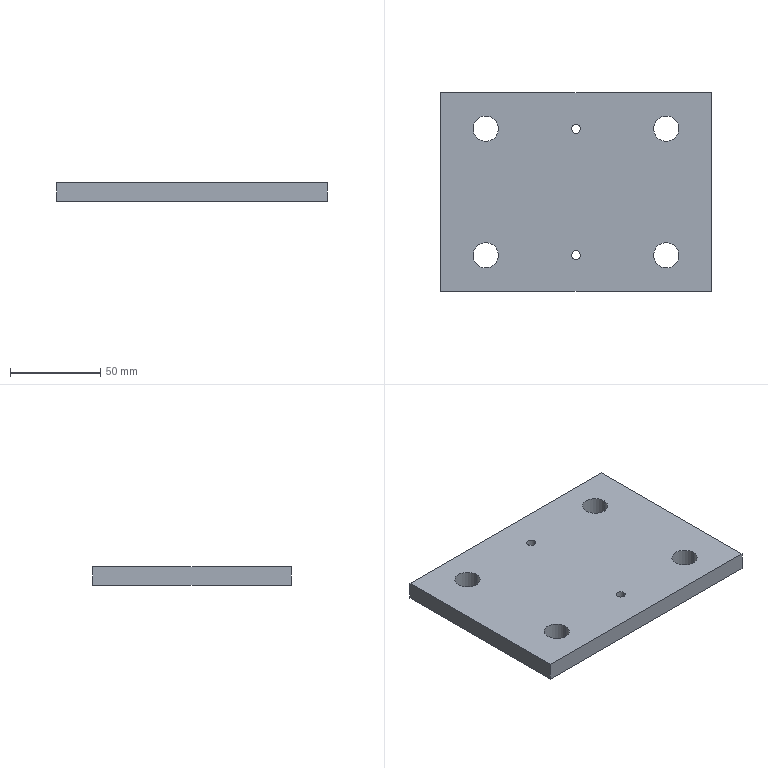Component | SolidWorks | THK-A1025ColumnFixingPlate-6 | 1 solid | 18 faces | box 150 x 110 x 10 mm | volume 158450 mm3 | cylinder 12 | plane 6 | commonest cylinder face diameters 14 x8 5 x4 | material Q235A
build123d program:
from build123d import *

# Parameters (mm, degrees)
SKETCH1_W                  = 150
SKETCH1_H                  = 110
BOSS_EXTRUDE1_DEPTH        = 5
F_14_0_14_DIAMETER_HOLE1_D = 14
M6_TAPPED_HOLE1_D          = 5


with BuildPart() as part:
    # Sketch1 → Boss-Extrude1 (new, symmetric)
    with BuildSketch(Plane.XY):
        Rectangle(SKETCH1_W, SKETCH1_H)
    extrude(amount=BOSS_EXTRUDE1_DEPTH, both=True)

    # 14.0 _14_ Diameter Hole1 (through all)
    with Locations(Plane.XY.offset(5)):
        with Locations((-50, 35), (50, 35), (50, -35), (-50, -35)):
            Hole(F_14_0_14_DIAMETER_HOLE1_D / 2)

    # M6 Tapped Hole1 (through all)
    with Locations(Plane.XY.offset(5)):
        with Locations((0, 35), (0, -35)):
            Hole(M6_TAPPED_HOLE1_D / 2)


solid = part.part

# Placed as in the assembly
solid = solid.moved(Location((0, 625, -376), (0, 0, 0)))
STEP:
#1=COLOUR_RGB('',0.7922,0.8196,0.9333);
#2=FILL_AREA_STYLE_COLOUR('',#1);
#3=FILL_AREA_STYLE('',(#2));
#4=SURFACE_STYLE_FILL_AREA(#3);
#5=SURFACE_SIDE_STYLE('',(#4));
#6=SURFACE_STYLE_USAGE(.BOTH.,#5);
#7=PRESENTATION_STYLE_ASSIGNMENT((#6));
#8=CARTESIAN_POINT('',(-0.09843,25.984,-15.));
#9=VERTEX_POINT('',#8);
#10=CARTESIAN_POINT('',(0.09843,25.984,-15.));
#11=VERTEX_POINT('',#10);
#12=CARTESIAN_POINT('',(0.,25.984,-15.));
#13=DIRECTION('',(0.,0.,1.));
#14=DIRECTION('',(1.,0.,0.));
#15=AXIS2_PLACEMENT_3D('',#12,#13,#14);
#16=CIRCLE('',#15,0.09843);
#17=EDGE_CURVE('',#9,#11,#16,.T.);
#18=ORIENTED_EDGE('',*,*,#17,.F.);
#19=CARTESIAN_POINT('',(-0.09843,25.984,-14.606));
#20=VERTEX_POINT('',#19);
#21=CARTESIAN_POINT('',(-0.09843,25.984,-14.606));
#22=DIRECTION('',(0.,0.,1.));
#23=VECTOR('',#22,39.37);
#24=LINE('',#21,#23);
#25=EDGE_CURVE('',#9,#20,#24,.T.);
#26=ORIENTED_EDGE('',*,*,#25,.T.);
#27=CARTESIAN_POINT('',(0.09843,25.984,-14.606));
#28=VERTEX_POINT('',#27);
#29=CARTESIAN_POINT('',(0.,25.984,-14.606));
#30=DIRECTION('',(0.,0.,1.));
#31=DIRECTION('',(1.,0.,0.));
#32=AXIS2_PLACEMENT_3D('',#29,#30,#31);
#33=CIRCLE('',#32,0.09843);
#34=EDGE_CURVE('',#20,#28,#33,.T.);
#35=ORIENTED_EDGE('',*,*,#34,.T.);
#36=CARTESIAN_POINT('',(0.09843,25.984,-14.606));
#37=DIRECTION('',(0.,0.,1.));
#38=VECTOR('',#37,39.37);
#39=LINE('',#36,#38);
#40=EDGE_CURVE('',#11,#28,#39,.T.);
#41=ORIENTED_EDGE('',*,*,#40,.F.);
#42=EDGE_LOOP('',(#18,#26,#35,#41));
#43=FACE_OUTER_BOUND('',#42,.T.);
#44=CARTESIAN_POINT('',(0.,25.984,-14.606));
#45=DIRECTION('',(0.,0.,1.));
#46=DIRECTION('',(1.,0.,0.));
#47=AXIS2_PLACEMENT_3D('',#44,#45,#46);
#48=CYLINDRICAL_SURFACE('',#47,0.09843);
#49=ADVANCED_FACE('',(#43),#48,.F.);
#50=CARTESIAN_POINT('',(-0.09843,23.228,-15.));
#51=VERTEX_POINT('',#50);
#52=CARTESIAN_POINT('',(0.09843,23.228,-15.));
#53=VERTEX_POINT('',#52);
#54=CARTESIAN_POINT('',(0.,23.228,-15.));
#55=DIRECTION('',(0.,0.,1.));
#56=DIRECTION('',(1.,0.,0.));
#57=AXIS2_PLACEMENT_3D('',#54,#55,#56);
#58=CIRCLE('',#57,0.09843);
#59=EDGE_CURVE('',#51,#53,#58,.T.);
#60=ORIENTED_EDGE('',*,*,#59,.F.);
#61=CARTESIAN_POINT('',(-0.09843,23.228,-14.606));
#62=VERTEX_POINT('',#61);
#63=CARTESIAN_POINT('',(-0.09843,23.228,-14.606));
#64=DIRECTION('',(0.,0.,1.));
#65=VECTOR('',#64,39.37);
#66=LINE('',#63,#65);
#67=EDGE_CURVE('',#51,#62,#66,.T.);
#68=ORIENTED_EDGE('',*,*,#67,.T.);
#69=CARTESIAN_POINT('',(0.09843,23.228,-14.606));
#70=VERTEX_POINT('',#69);
#71=CARTESIAN_POINT('',(0.,23.228,-14.606));
#72=DIRECTION('',(0.,0.,1.));
#73=DIRECTION('',(1.,0.,0.));
#74=AXIS2_PLACEMENT_3D('',#71,#72,#73);
#75=CIRCLE('',#74,0.09843);
#76=EDGE_CURVE('',#62,#70,#75,.T.);
#77=ORIENTED_EDGE('',*,*,#76,.T.);
#78=CARTESIAN_POINT('',(0.09843,23.228,-14.606));
#79=DIRECTION('',(0.,0.,1.));
#80=VECTOR('',#79,39.37);
#81=LINE('',#78,#80);
#82=EDGE_CURVE('',#53,#70,#81,.T.);
#83=ORIENTED_EDGE('',*,*,#82,.F.);
#84=EDGE_LOOP('',(#60,#68,#77,#83));
#85=FACE_OUTER_BOUND('',#84,.T.);
#86=CARTESIAN_POINT('',(0.,23.228,-14.606));
#87=DIRECTION('',(0.,0.,1.));
#88=DIRECTION('',(1.,0.,0.));
#89=AXIS2_PLACEMENT_3D('',#86,#87,#88);
#90=CYLINDRICAL_SURFACE('',#89,0.09843);
#91=ADVANCED_FACE('',(#85),#90,.F.);
#92=CARTESIAN_POINT('',(-2.244,25.984,-15.));
#93=VERTEX_POINT('',#92);
#94=CARTESIAN_POINT('',(-1.693,25.984,-15.));
#95=VERTEX_POINT('',#94);
#96=CARTESIAN_POINT('',(-1.969,25.984,-15.));
#97=DIRECTION('',(0.,0.,1.));
#98=DIRECTION('',(1.,0.,0.));
#99=AXIS2_PLACEMENT_3D('',#96,#97,#98);
#100=CIRCLE('',#99,0.2756);
#101=EDGE_CURVE('',#93,#95,#100,.T.);
#102=ORIENTED_EDGE('',*,*,#101,.F.);
#103=CARTESIAN_POINT('',(-2.244,25.984,-14.606));
#104=VERTEX_POINT('',#103);
#105=CARTESIAN_POINT('',(-2.244,25.984,-14.606));
#106=DIRECTION('',(0.,0.,1.));
#107=VECTOR('',#106,39.37);
#108=LINE('',#105,#107);
#109=EDGE_CURVE('',#93,#104,#108,.T.);
#110=ORIENTED_EDGE('',*,*,#109,.T.);
#111=CARTESIAN_POINT('',(-1.693,25.984,-14.606));
#112=VERTEX_POINT('',#111);
#113=CARTESIAN_POINT('',(-1.969,25.984,-14.606));
#114=DIRECTION('',(0.,0.,1.));
#115=DIRECTION('',(1.,0.,0.));
#116=AXIS2_PLACEMENT_3D('',#113,#114,#115);
#117=CIRCLE('',#116,0.2756);
#118=EDGE_CURVE('',#104,#112,#117,.T.);
#119=ORIENTED_EDGE('',*,*,#118,.T.);
#120=CARTESIAN_POINT('',(-1.693,25.984,-14.606));
#121=DIRECTION('',(0.,0.,1.));
#122=VECTOR('',#121,39.37);
#123=LINE('',#120,#122);
#124=EDGE_CURVE('',#95,#112,#123,.T.);
#125=ORIENTED_EDGE('',*,*,#124,.F.);
#126=EDGE_LOOP('',(#102,#110,#119,#125));
#127=FACE_OUTER_BOUND('',#126,.T.);
#128=CARTESIAN_POINT('',(-1.969,25.984,-14.606));
#129=DIRECTION('',(0.,0.,1.));
#130=DIRECTION('',(1.,0.,0.));
#131=AXIS2_PLACEMENT_3D('',#128,#129,#130);
#132=CYLINDRICAL_SURFACE('',#131,0.2756);
#133=ADVANCED_FACE('',(#127),#132,.F.);
#134=CARTESIAN_POINT('',(1.693,25.984,-15.));
#135=VERTEX_POINT('',#134);
#136=CARTESIAN_POINT('',(2.244,25.984,-15.));
#137=VERTEX_POINT('',#136);
#138=CARTESIAN_POINT('',(1.969,25.984,-15.));
#139=DIRECTION('',(0.,0.,1.));
#140=DIRECTION('',(1.,0.,0.));
#141=AXIS2_PLACEMENT_3D('',#138,#139,#140);
#142=CIRCLE('',#141,0.2756);
#143=EDGE_CURVE('',#135,#137,#142,.T.);
#144=ORIENTED_EDGE('',*,*,#143,.F.);
#145=CARTESIAN_POINT('',(1.693,25.984,-14.606));
#146=VERTEX_POINT('',#145);
#147=CARTESIAN_POINT('',(1.693,25.984,-14.606));
#148=DIRECTION('',(0.,0.,1.));
#149=VECTOR('',#148,39.37);
#150=LINE('',#147,#149);
#151=EDGE_CURVE('',#135,#146,#150,.T.);
#152=ORIENTED_EDGE('',*,*,#151,.T.);
#153=CARTESIAN_POINT('',(2.244,25.984,-14.606));
#154=VERTEX_POINT('',#153);
#155=CARTESIAN_POINT('',(1.969,25.984,-14.606));
#156=DIRECTION('',(0.,0.,1.));
#157=DIRECTION('',(1.,0.,0.));
#158=AXIS2_PLACEMENT_3D('',#155,#156,#157);
#159=CIRCLE('',#158,0.2756);
#160=EDGE_CURVE('',#146,#154,#159,.T.);
#161=ORIENTED_EDGE('',*,*,#160,.T.);
#162=CARTESIAN_POINT('',(2.244,25.984,-14.606));
#163=DIRECTION('',(0.,0.,1.));
#164=VECTOR('',#163,39.37);
#165=LINE('',#162,#164);
#166=EDGE_CURVE('',#137,#154,#165,.T.);
#167=ORIENTED_EDGE('',*,*,#166,.F.);
#168=EDGE_LOOP('',(#144,#152,#161,#167));
#169=FACE_OUTER_BOUND('',#168,.T.);
#170=CARTESIAN_POINT('',(1.969,25.984,-14.606));
#171=DIRECTION('',(0.,0.,1.));
#172=DIRECTION('',(1.,0.,0.));
#173=AXIS2_PLACEMENT_3D('',#170,#171,#172);
#174=CYLINDRICAL_SURFACE('',#173,0.2756);
#175=ADVANCED_FACE('',(#169),#174,.F.);
#176=CARTESIAN_POINT('',(1.693,23.228,-15.));
#177=VERTEX_POINT('',#176);
#178=CARTESIAN_POINT('',(2.244,23.228,-15.));
#179=VERTEX_POINT('',#178);
#180=CARTESIAN_POINT('',(1.969,23.228,-15.));
#181=DIRECTION('',(0.,0.,1.));
#182=DIRECTION('',(1.,0.,0.));
#183=AXIS2_PLACEMENT_3D('',#180,#181,#182);
#184=CIRCLE('',#183,0.2756);
#185=EDGE_CURVE('',#177,#179,#184,.T.);
#186=ORIENTED_EDGE('',*,*,#185,.F.);
#187=CARTESIAN_POINT('',(1.693,23.228,-14.606));
#188=VERTEX_POINT('',#187);
#189=CARTESIAN_POINT('',(1.693,23.228,-14.606));
#190=DIRECTION('',(0.,0.,1.));
#191=VECTOR('',#190,39.37);
#192=LINE('',#189,#191);
#193=EDGE_CURVE('',#177,#188,#192,.T.);
#194=ORIENTED_EDGE('',*,*,#193,.T.);
#195=CARTESIAN_POINT('',(2.244,23.228,-14.606));
#196=VERTEX_POINT('',#195);
#197=CARTESIAN_POINT('',(1.969,23.228,-14.606));
#198=DIRECTION('',(0.,0.,1.));
#199=DIRECTION('',(1.,0.,0.));
#200=AXIS2_PLACEMENT_3D('',#197,#198,#199);
#201=CIRCLE('',#200,0.2756);
#202=EDGE_CURVE('',#188,#196,#201,.T.);
#203=ORIENTED_EDGE('',*,*,#202,.T.);
#204=CARTESIAN_POINT('',(2.244,23.228,-14.606));
#205=DIRECTION('',(0.,0.,1.));
#206=VECTOR('',#205,39.37);
#207=LINE('',#204,#206);
#208=EDGE_CURVE('',#179,#196,#207,.T.);
#209=ORIENTED_EDGE('',*,*,#208,.F.);
#210=EDGE_LOOP('',(#186,#194,#203,#209));
#211=FACE_OUTER_BOUND('',#210,.T.);
#212=CARTESIAN_POINT('',(1.969,23.228,-14.606));
#213=DIRECTION('',(0.,0.,1.));
#214=DIRECTION('',(1.,0.,0.));
#215=AXIS2_PLACEMENT_3D('',#212,#213,#214);
#216=CYLINDRICAL_SURFACE('',#215,0.2756);
#217=ADVANCED_FACE('',(#211),#216,.F.);
#218=CARTESIAN_POINT('',(-2.244,23.228,-15.));
#219=VERTEX_POINT('',#218);
#220=CARTESIAN_POINT('',(-1.693,23.228,-15.));
#221=VERTEX_POINT('',#220);
#222=CARTESIAN_POINT('',(-1.969,23.228,-15.));
#223=DIRECTION('',(0.,0.,1.));
#224=DIRECTION('',(1.,0.,0.));
#225=AXIS2_PLACEMENT_3D('',#222,#223,#224);
#226=CIRCLE('',#225,0.2756);
#227=EDGE_CURVE('',#219,#221,#226,.T.);
#228=ORIENTED_EDGE('',*,*,#227,.F.);
#229=CARTESIAN_POINT('',(-2.244,23.228,-14.606));
#230=VERTEX_POINT('',#229);
#231=CARTESIAN_POINT('',(-2.244,23.228,-14.606));
#232=DIRECTION('',(0.,0.,1.));
#233=VECTOR('',#232,39.37);
#234=LINE('',#231,#233);
#235=EDGE_CURVE('',#219,#230,#234,.T.);
#236=ORIENTED_EDGE('',*,*,#235,.T.);
#237=CARTESIAN_POINT('',(-1.693,23.228,-14.606));
#238=VERTEX_POINT('',#237);
#239=CARTESIAN_POINT('',(-1.969,23.228,-14.606));
#240=DIRECTION('',(0.,0.,1.));
#241=DIRECTION('',(1.,0.,0.));
#242=AXIS2_PLACEMENT_3D('',#239,#240,#241);
#243=CIRCLE('',#242,0.2756);
#244=EDGE_CURVE('',#230,#238,#243,.T.);
#245=ORIENTED_EDGE('',*,*,#244,.T.);
#246=CARTESIAN_POINT('',(-1.693,23.228,-14.606));
#247=DIRECTION('',(0.,0.,1.));
#248=VECTOR('',#247,39.37);
#249=LINE('',#246,#248);
#250=EDGE_CURVE('',#221,#238,#249,.T.);
#251=ORIENTED_EDGE('',*,*,#250,.F.);
#252=EDGE_LOOP('',(#228,#236,#245,#251));
#253=FACE_OUTER_BOUND('',#252,.T.);
#254=CARTESIAN_POINT('',(-1.969,23.228,-14.606));
#255=DIRECTION('',(0.,0.,1.));
#256=DIRECTION('',(1.,0.,0.));
#257=AXIS2_PLACEMENT_3D('',#254,#255,#256);
#258=CYLINDRICAL_SURFACE('',#257,0.2756);
#259=ADVANCED_FACE('',(#253),#258,.F.);
#260=CARTESIAN_POINT('',(2.953,22.441,-15.));
#261=VERTEX_POINT('',#260);
#262=CARTESIAN_POINT('',(2.953,26.772,-15.));
#263=VERTEX_POINT('',#262);
#264=CARTESIAN_POINT('',(2.953,22.441,-15.));
#265=DIRECTION('',(0.,1.,0.));
#266=VECTOR('',#265,39.37);
#267=LINE('',#264,#266);
#268=EDGE_CURVE('',#261,#263,#267,.T.);
#269=ORIENTED_EDGE('',*,*,#268,.T.);
#270=CARTESIAN_POINT('',(2.953,26.772,-14.606));
#271=VERTEX_POINT('',#270);
#272=CARTESIAN_POINT('',(2.953,26.772,-14.606));
#273=DIRECTION('',(0.,0.,-1.));
#274=VECTOR('',#273,39.37);
#275=LINE('',#272,#274);
#276=EDGE_CURVE('',#271,#263,#275,.T.);
#277=ORIENTED_EDGE('',*,*,#276,.F.);
#278=CARTESIAN_POINT('',(2.953,22.441,-14.606));
#279=VERTEX_POINT('',#278);
#280=CARTESIAN_POINT('',(2.953,22.441,-14.606));
#281=DIRECTION('',(0.,1.,0.));
#282=VECTOR('',#281,39.37);
#283=LINE('',#280,#282);
#284=EDGE_CURVE('',#279,#271,#283,.T.);
#285=ORIENTED_EDGE('',*,*,#284,.F.);
#286=CARTESIAN_POINT('',(2.953,22.441,-14.606));
#287=DIRECTION('',(0.,0.,-1.));
#288=VECTOR('',#287,39.37);
#289=LINE('',#286,#288);
#290=EDGE_CURVE('',#279,#261,#289,.T.);
#291=ORIENTED_EDGE('',*,*,#290,.T.);
#292=EDGE_LOOP('',(#269,#277,#285,#291));
#293=FACE_OUTER_BOUND('',#292,.T.);
#294=CARTESIAN_POINT('',(2.953,22.441,-14.606));
#295=DIRECTION('',(-1.,0.,0.));
#296=DIRECTION('',(0.,0.,1.));
#297=AXIS2_PLACEMENT_3D('',#294,#295,#296);
#298=PLANE('',#297);
#299=ADVANCED_FACE('',(#293),#298,.F.);
#300=CARTESIAN_POINT('',(-2.953,26.772,-15.));
#301=VERTEX_POINT('',#300);
#302=CARTESIAN_POINT('',(-2.953,26.772,-15.));
#303=DIRECTION('',(-1.,0.,0.));
#304=VECTOR('',#303,39.37);
#305=LINE('',#302,#304);
#306=EDGE_CURVE('',#263,#301,#305,.T.);
#307=ORIENTED_EDGE('',*,*,#306,.T.);
#308=CARTESIAN_POINT('',(-2.953,26.772,-14.606));
#309=VERTEX_POINT('',#308);
#310=CARTESIAN_POINT('',(-2.953,26.772,-14.606));
#311=DIRECTION('',(0.,0.,-1.));
#312=VECTOR('',#311,39.37);
#313=LINE('',#310,#312);
#314=EDGE_CURVE('',#309,#301,#313,.T.);
#315=ORIENTED_EDGE('',*,*,#314,.F.);
#316=CARTESIAN_POINT('',(-2.953,26.772,-14.606));
#317=DIRECTION('',(-1.,0.,0.));
#318=VECTOR('',#317,39.37);
#319=LINE('',#316,#318);
#320=EDGE_CURVE('',#271,#309,#319,.T.);
#321=ORIENTED_EDGE('',*,*,#320,.F.);
#322=ORIENTED_EDGE('',*,*,#276,.T.);
#323=EDGE_LOOP('',(#307,#315,#321,#322));
#324=FACE_OUTER_BOUND('',#323,.T.);
#325=CARTESIAN_POINT('',(-2.953,26.772,-14.606));
#326=DIRECTION('',(0.,-1.,0.));
#327=DIRECTION('',(0.,0.,-1.));
#328=AXIS2_PLACEMENT_3D('',#325,#326,#327);
#329=PLANE('',#328);
#330=ADVANCED_FACE('',(#324),#329,.F.);
#331=CARTESIAN_POINT('',(-2.953,22.441,-15.));
#332=VERTEX_POINT('',#331);
#333=CARTESIAN_POINT('',(-2.953,22.441,-15.));
#334=DIRECTION('',(0.,-1.,0.));
#335=VECTOR('',#334,39.37);
#336=LINE('',#333,#335);
#337=EDGE_CURVE('',#301,#332,#336,.T.);
#338=ORIENTED_EDGE('',*,*,#337,.T.);
#339=CARTESIAN_POINT('',(-2.953,22.441,-14.606));
#340=VERTEX_POINT('',#339);
#341=CARTESIAN_POINT('',(-2.953,22.441,-14.606));
#342=DIRECTION('',(0.,0.,-1.));
#343=VECTOR('',#342,39.37);
#344=LINE('',#341,#343);
#345=EDGE_CURVE('',#340,#332,#344,.T.);
#346=ORIENTED_EDGE('',*,*,#345,.F.);
#347=CARTESIAN_POINT('',(-2.953,22.441,-14.606));
#348=DIRECTION('',(0.,-1.,0.));
#349=VECTOR('',#348,39.37);
#350=LINE('',#347,#349);
#351=EDGE_CURVE('',#309,#340,#350,.T.);
#352=ORIENTED_EDGE('',*,*,#351,.F.);
#353=ORIENTED_EDGE('',*,*,#314,.T.);
#354=EDGE_LOOP('',(#338,#346,#352,#353));
#355=FACE_OUTER_BOUND('',#354,.T.);
#356=CARTESIAN_POINT('',(-2.953,22.441,-14.606));
#357=DIRECTION('',(1.,0.,0.));
#358=DIRECTION('',(0.,0.,-1.));
#359=AXIS2_PLACEMENT_3D('',#356,#357,#358);
#360=PLANE('',#359);
#361=ADVANCED_FACE('',(#355),#360,.F.);
#362=CARTESIAN_POINT('',(-2.953,22.441,-15.));
#363=DIRECTION('',(1.,0.,0.));
#364=VECTOR('',#363,39.37);
#365=LINE('',#362,#364);
#366=EDGE_CURVE('',#332,#261,#365,.T.);
#367=ORIENTED_EDGE('',*,*,#366,.T.);
#368=ORIENTED_EDGE('',*,*,#290,.F.);
#369=CARTESIAN_POINT('',(-2.953,22.441,-14.606));
#370=DIRECTION('',(1.,0.,0.));
#371=VECTOR('',#370,39.37);
#372=LINE('',#369,#371);
#373=EDGE_CURVE('',#340,#279,#372,.T.);
#374=ORIENTED_EDGE('',*,*,#373,.F.);
#375=ORIENTED_EDGE('',*,*,#345,.T.);
#376=EDGE_LOOP('',(#367,#368,#374,#375));
#377=FACE_OUTER_BOUND('',#376,.T.);
#378=CARTESIAN_POINT('',(-2.953,22.441,-14.606));
#379=DIRECTION('',(0.,1.,0.));
#380=DIRECTION('',(0.,0.,1.));
#381=AXIS2_PLACEMENT_3D('',#378,#379,#380);
#382=PLANE('',#381);
#383=ADVANCED_FACE('',(#377),#382,.F.);
#384=CARTESIAN_POINT('',(0.,25.984,-14.606));
#385=DIRECTION('',(0.,0.,1.));
#386=DIRECTION('',(1.,0.,0.));
#387=AXIS2_PLACEMENT_3D('',#384,#385,#386);
#388=CIRCLE('',#387,0.09843);
#389=EDGE_CURVE('',#28,#20,#388,.T.);
#390=ORIENTED_EDGE('',*,*,#389,.F.);
#391=ORIENTED_EDGE('',*,*,#34,.F.);
#392=EDGE_LOOP('',(#390,#391));
#393=FACE_BOUND('',#392,.T.);
#394=CARTESIAN_POINT('',(0.,23.228,-14.606));
#395=DIRECTION('',(0.,0.,1.));
#396=DIRECTION('',(1.,0.,0.));
#397=AXIS2_PLACEMENT_3D('',#394,#395,#396);
#398=CIRCLE('',#397,0.09843);
#399=EDGE_CURVE('',#70,#62,#398,.T.);
#400=ORIENTED_EDGE('',*,*,#399,.F.);
#401=ORIENTED_EDGE('',*,*,#76,.F.);
#402=EDGE_LOOP('',(#400,#401));
#403=FACE_BOUND('',#402,.T.);
#404=CARTESIAN_POINT('',(-1.969,25.984,-14.606));
#405=DIRECTION('',(0.,0.,1.));
#406=DIRECTION('',(1.,0.,0.));
#407=AXIS2_PLACEMENT_3D('',#404,#405,#406);
#408=CIRCLE('',#407,0.2756);
#409=EDGE_CURVE('',#112,#104,#408,.T.);
#410=ORIENTED_EDGE('',*,*,#409,.F.);
#411=ORIENTED_EDGE('',*,*,#118,.F.);
#412=EDGE_LOOP('',(#410,#411));
#413=FACE_BOUND('',#412,.T.);
#414=CARTESIAN_POINT('',(1.969,25.984,-14.606));
#415=DIRECTION('',(0.,0.,1.));
#416=DIRECTION('',(1.,0.,0.));
#417=AXIS2_PLACEMENT_3D('',#414,#415,#416);
#418=CIRCLE('',#417,0.2756);
#419=EDGE_CURVE('',#154,#146,#418,.T.);
#420=ORIENTED_EDGE('',*,*,#419,.F.);
#421=ORIENTED_EDGE('',*,*,#160,.F.);
#422=EDGE_LOOP('',(#420,#421));
#423=FACE_BOUND('',#422,.T.);
#424=CARTESIAN_POINT('',(1.969,23.228,-14.606));
#425=DIRECTION('',(0.,0.,1.));
#426=DIRECTION('',(1.,0.,0.));
#427=AXIS2_PLACEMENT_3D('',#424,#425,#426);
#428=CIRCLE('',#427,0.2756);
#429=EDGE_CURVE('',#196,#188,#428,.T.);
#430=ORIENTED_EDGE('',*,*,#429,.F.);
#431=ORIENTED_EDGE('',*,*,#202,.F.);
#432=EDGE_LOOP('',(#430,#431));
#433=FACE_BOUND('',#432,.T.);
#434=CARTESIAN_POINT('',(-1.969,23.228,-14.606));
#435=DIRECTION('',(0.,0.,1.));
#436=DIRECTION('',(1.,0.,0.));
#437=AXIS2_PLACEMENT_3D('',#434,#435,#436);
#438=CIRCLE('',#437,0.2756);
#439=EDGE_CURVE('',#238,#230,#438,.T.);
#440=ORIENTED_EDGE('',*,*,#439,.F.);
#441=ORIENTED_EDGE('',*,*,#244,.F.);
#442=EDGE_LOOP('',(#440,#441));
#443=FACE_BOUND('',#442,.T.);
#444=ORIENTED_EDGE('',*,*,#284,.T.);
#445=ORIENTED_EDGE('',*,*,#320,.T.);
#446=ORIENTED_EDGE('',*,*,#351,.T.);
#447=ORIENTED_EDGE('',*,*,#373,.T.);
#448=EDGE_LOOP('',(#444,#445,#446,#447));
#449=FACE_OUTER_BOUND('',#448,.T.);
#450=CARTESIAN_POINT('',(0.,24.606,-14.606));
#451=DIRECTION('',(0.,0.,-1.));
#452=DIRECTION('',(-1.,0.,0.));
#453=AXIS2_PLACEMENT_3D('',#450,#451,#452);
#454=PLANE('',#453);
#455=ADVANCED_FACE('',(#393,#403,#413,#423,#433,#443,#449),#454,.F.);
#456=CARTESIAN_POINT('',(0.,25.984,-15.));
#457=DIRECTION('',(0.,0.,1.));
#458=DIRECTION('',(1.,0.,0.));
#459=AXIS2_PLACEMENT_3D('',#456,#457,#458);
#460=CIRCLE('',#459,0.09843);
#461=EDGE_CURVE('',#11,#9,#460,.T.);
#462=ORIENTED_EDGE('',*,*,#461,.T.);
#463=ORIENTED_EDGE('',*,*,#17,.T.);
#464=EDGE_LOOP('',(#462,#463));
#465=FACE_BOUND('',#464,.T.);
#466=CARTESIAN_POINT('',(0.,23.228,-15.));
#467=DIRECTION('',(0.,0.,1.));
#468=DIRECTION('',(1.,0.,0.));
#469=AXIS2_PLACEMENT_3D('',#466,#467,#468);
#470=CIRCLE('',#469,0.09843);
#471=EDGE_CURVE('',#53,#51,#470,.T.);
#472=ORIENTED_EDGE('',*,*,#471,.T.);
#473=ORIENTED_EDGE('',*,*,#59,.T.);
#474=EDGE_LOOP('',(#472,#473));
#475=FACE_BOUND('',#474,.T.);
#476=CARTESIAN_POINT('',(-1.969,25.984,-15.));
#477=DIRECTION('',(0.,0.,1.));
#478=DIRECTION('',(1.,0.,0.));
#479=AXIS2_PLACEMENT_3D('',#476,#477,#478);
#480=CIRCLE('',#479,0.2756);
#481=EDGE_CURVE('',#95,#93,#480,.T.);
#482=ORIENTED_EDGE('',*,*,#481,.T.);
#483=ORIENTED_EDGE('',*,*,#101,.T.);
#484=EDGE_LOOP('',(#482,#483));
#485=FACE_BOUND('',#484,.T.);
#486=CARTESIAN_POINT('',(1.969,25.984,-15.));
#487=DIRECTION('',(0.,0.,1.));
#488=DIRECTION('',(1.,0.,0.));
#489=AXIS2_PLACEMENT_3D('',#486,#487,#488);
#490=CIRCLE('',#489,0.2756);
#491=EDGE_CURVE('',#137,#135,#490,.T.);
#492=ORIENTED_EDGE('',*,*,#491,.T.);
#493=ORIENTED_EDGE('',*,*,#143,.T.);
#494=EDGE_LOOP('',(#492,#493));
#495=FACE_BOUND('',#494,.T.);
#496=CARTESIAN_POINT('',(1.969,23.228,-15.));
#497=DIRECTION('',(0.,0.,1.));
#498=DIRECTION('',(1.,0.,0.));
#499=AXIS2_PLACEMENT_3D('',#496,#497,#498);
#500=CIRCLE('',#499,0.2756);
#501=EDGE_CURVE('',#179,#177,#500,.T.);
#502=ORIENTED_EDGE('',*,*,#501,.T.);
#503=ORIENTED_EDGE('',*,*,#185,.T.);
#504=EDGE_LOOP('',(#502,#503));
#505=FACE_BOUND('',#504,.T.);
#506=CARTESIAN_POINT('',(-1.969,23.228,-15.));
#507=DIRECTION('',(0.,0.,1.));
#508=DIRECTION('',(1.,0.,0.));
#509=AXIS2_PLACEMENT_3D('',#506,#507,#508);
#510=CIRCLE('',#509,0.2756);
#511=EDGE_CURVE('',#221,#219,#510,.T.);
#512=ORIENTED_EDGE('',*,*,#511,.T.);
#513=ORIENTED_EDGE('',*,*,#227,.T.);
#514=EDGE_LOOP('',(#512,#513));
#515=FACE_BOUND('',#514,.T.);
#516=ORIENTED_EDGE('',*,*,#268,.F.);
#517=ORIENTED_EDGE('',*,*,#366,.F.);
#518=ORIENTED_EDGE('',*,*,#337,.F.);
#519=ORIENTED_EDGE('',*,*,#306,.F.);
#520=EDGE_LOOP('',(#516,#517,#518,#519));
#521=FACE_OUTER_BOUND('',#520,.T.);
#522=CARTESIAN_POINT('',(0.,24.606,-15.));
#523=DIRECTION('',(0.,0.,-1.));
#524=DIRECTION('',(-1.,0.,0.));
#525=AXIS2_PLACEMENT_3D('',#522,#523,#524);
#526=PLANE('',#525);
#527=ADVANCED_FACE('',(#465,#475,#485,#495,#505,#515,#521),#526,.T.);
#528=ORIENTED_EDGE('',*,*,#235,.F.);
#529=ORIENTED_EDGE('',*,*,#511,.F.);
#530=ORIENTED_EDGE('',*,*,#250,.T.);
#531=ORIENTED_EDGE('',*,*,#439,.T.);
#532=EDGE_LOOP('',(#528,#529,#530,#531));
#533=FACE_OUTER_BOUND('',#532,.T.);
#534=CARTESIAN_POINT('',(-1.969,23.228,-14.606));
#535=DIRECTION('',(0.,0.,1.));
#536=DIRECTION('',(1.,0.,0.));
#537=AXIS2_PLACEMENT_3D('',#534,#535,#536);
#538=CYLINDRICAL_SURFACE('',#537,0.2756);
#539=ADVANCED_FACE('',(#533),#538,.F.);
#540=ORIENTED_EDGE('',*,*,#193,.F.);
#541=ORIENTED_EDGE('',*,*,#501,.F.);
#542=ORIENTED_EDGE('',*,*,#208,.T.);
#543=ORIENTED_EDGE('',*,*,#429,.T.);
#544=EDGE_LOOP('',(#540,#541,#542,#543));
#545=FACE_OUTER_BOUND('',#544,.T.);
#546=CARTESIAN_POINT('',(1.969,23.228,-14.606));
#547=DIRECTION('',(0.,0.,1.));
#548=DIRECTION('',(1.,0.,0.));
#549=AXIS2_PLACEMENT_3D('',#546,#547,#548);
#550=CYLINDRICAL_SURFACE('',#549,0.2756);
#551=ADVANCED_FACE('',(#545),#550,.F.);
#552=ORIENTED_EDGE('',*,*,#151,.F.);
#553=ORIENTED_EDGE('',*,*,#491,.F.);
#554=ORIENTED_EDGE('',*,*,#166,.T.);
#555=ORIENTED_EDGE('',*,*,#419,.T.);
#556=EDGE_LOOP('',(#552,#553,#554,#555));
#557=FACE_OUTER_BOUND('',#556,.T.);
#558=CARTESIAN_POINT('',(1.969,25.984,-14.606));
#559=DIRECTION('',(0.,0.,1.));
#560=DIRECTION('',(1.,0.,0.));
#561=AXIS2_PLACEMENT_3D('',#558,#559,#560);
#562=CYLINDRICAL_SURFACE('',#561,0.2756);
#563=ADVANCED_FACE('',(#557),#562,.F.);
#564=ORIENTED_EDGE('',*,*,#109,.F.);
#565=ORIENTED_EDGE('',*,*,#481,.F.);
#566=ORIENTED_EDGE('',*,*,#124,.T.);
#567=ORIENTED_EDGE('',*,*,#409,.T.);
#568=EDGE_LOOP('',(#564,#565,#566,#567));
#569=FACE_OUTER_BOUND('',#568,.T.);
#570=CARTESIAN_POINT('',(-1.969,25.984,-14.606));
#571=DIRECTION('',(0.,0.,1.));
#572=DIRECTION('',(1.,0.,0.));
#573=AXIS2_PLACEMENT_3D('',#570,#571,#572);
#574=CYLINDRICAL_SURFACE('',#573,0.2756);
#575=ADVANCED_FACE('',(#569),#574,.F.);
#576=ORIENTED_EDGE('',*,*,#67,.F.);
#577=ORIENTED_EDGE('',*,*,#471,.F.);
#578=ORIENTED_EDGE('',*,*,#82,.T.);
#579=ORIENTED_EDGE('',*,*,#399,.T.);
#580=EDGE_LOOP('',(#576,#577,#578,#579));
#581=FACE_OUTER_BOUND('',#580,.T.);
#582=CARTESIAN_POINT('',(0.,23.228,-14.606));
#583=DIRECTION('',(0.,0.,1.));
#584=DIRECTION('',(1.,0.,0.));
#585=AXIS2_PLACEMENT_3D('',#582,#583,#584);
#586=CYLINDRICAL_SURFACE('',#585,0.09843);
#587=ADVANCED_FACE('',(#581),#586,.F.);
#588=ORIENTED_EDGE('',*,*,#25,.F.);
#589=ORIENTED_EDGE('',*,*,#461,.F.);
#590=ORIENTED_EDGE('',*,*,#40,.T.);
#591=ORIENTED_EDGE('',*,*,#389,.T.);
#592=EDGE_LOOP('',(#588,#589,#590,#591));
#593=FACE_OUTER_BOUND('',#592,.T.);
#594=CARTESIAN_POINT('',(0.,25.984,-14.606));
#595=DIRECTION('',(0.,0.,1.));
#596=DIRECTION('',(1.,0.,0.));
#597=AXIS2_PLACEMENT_3D('',#594,#595,#596);
#598=CYLINDRICAL_SURFACE('',#597,0.09843);
#599=ADVANCED_FACE('',(#593),#598,.F.);
#600=CLOSED_SHELL('',(#49,#91,#133,#175,#217,#259,#299,#330,#361,#383,#455,#527,#539,#551,#563,#575,#587,#599));
#601=MANIFOLD_SOLID_BREP('',#600);
#602=STYLED_ITEM('',(#7),#601);
#603=PRESENTATION_LAYER_ASSIGNMENT('','',(#602));
#604=(LENGTH_UNIT()NAMED_UNIT(*)SI_UNIT($,.METRE.));
#605=LENGTH_MEASURE_WITH_UNIT(LENGTH_MEASURE(0.0254),#604);
#606=DIMENSIONAL_EXPONENTS(1.,0.,0.,0.,0.,0.,0.);
#607=(CONVERSION_BASED_UNIT('',#605)LENGTH_UNIT()NAMED_UNIT(#606));
#608=UNCERTAINTY_MEASURE_WITH_UNIT(LENGTH_MEASURE(0.00001),#607,'','');
#609=(NAMED_UNIT(*)PLANE_ANGLE_UNIT()SI_UNIT($,.RADIAN.));
#610=(NAMED_UNIT(*)SI_UNIT($,.STERADIAN.)SOLID_ANGLE_UNIT());
#611=(GEOMETRIC_REPRESENTATION_CONTEXT(3)GLOBAL_UNCERTAINTY_ASSIGNED_CONTEXT((#608))GLOBAL_UNIT_ASSIGNED_CONTEXT((#607,#609,#610))REPRESENTATION_CONTEXT('',''));
#612=MECHANICAL_DESIGN_GEOMETRIC_PRESENTATION_REPRESENTATION('',(#602),#611);
#613=CARTESIAN_POINT('',(0.,0.,0.));
#614=DIRECTION('',(0.,0.,1.));
#615=DIRECTION('',(1.,0.,0.));
#616=AXIS2_PLACEMENT_3D('',#613,#614,#615);
#617=(LENGTH_UNIT()NAMED_UNIT(*)SI_UNIT($,.METRE.));
#618=LENGTH_MEASURE_WITH_UNIT(LENGTH_MEASURE(0.0254),#617);
#619=DIMENSIONAL_EXPONENTS(1.,0.,0.,0.,0.,0.,0.);
#620=(CONVERSION_BASED_UNIT('',#618)LENGTH_UNIT()NAMED_UNIT(#619));
#621=UNCERTAINTY_MEASURE_WITH_UNIT(LENGTH_MEASURE(0.00001),#620,'','');
#622=(NAMED_UNIT(*)PLANE_ANGLE_UNIT()SI_UNIT($,.RADIAN.));
#623=(NAMED_UNIT(*)SI_UNIT($,.STERADIAN.)SOLID_ANGLE_UNIT());
#624=(GEOMETRIC_REPRESENTATION_CONTEXT(3)GLOBAL_UNCERTAINTY_ASSIGNED_CONTEXT((#621))GLOBAL_UNIT_ASSIGNED_CONTEXT((#620,#622,#623))REPRESENTATION_CONTEXT('',''));
#625=ADVANCED_BREP_SHAPE_REPRESENTATION('',(#601,#616),#624);